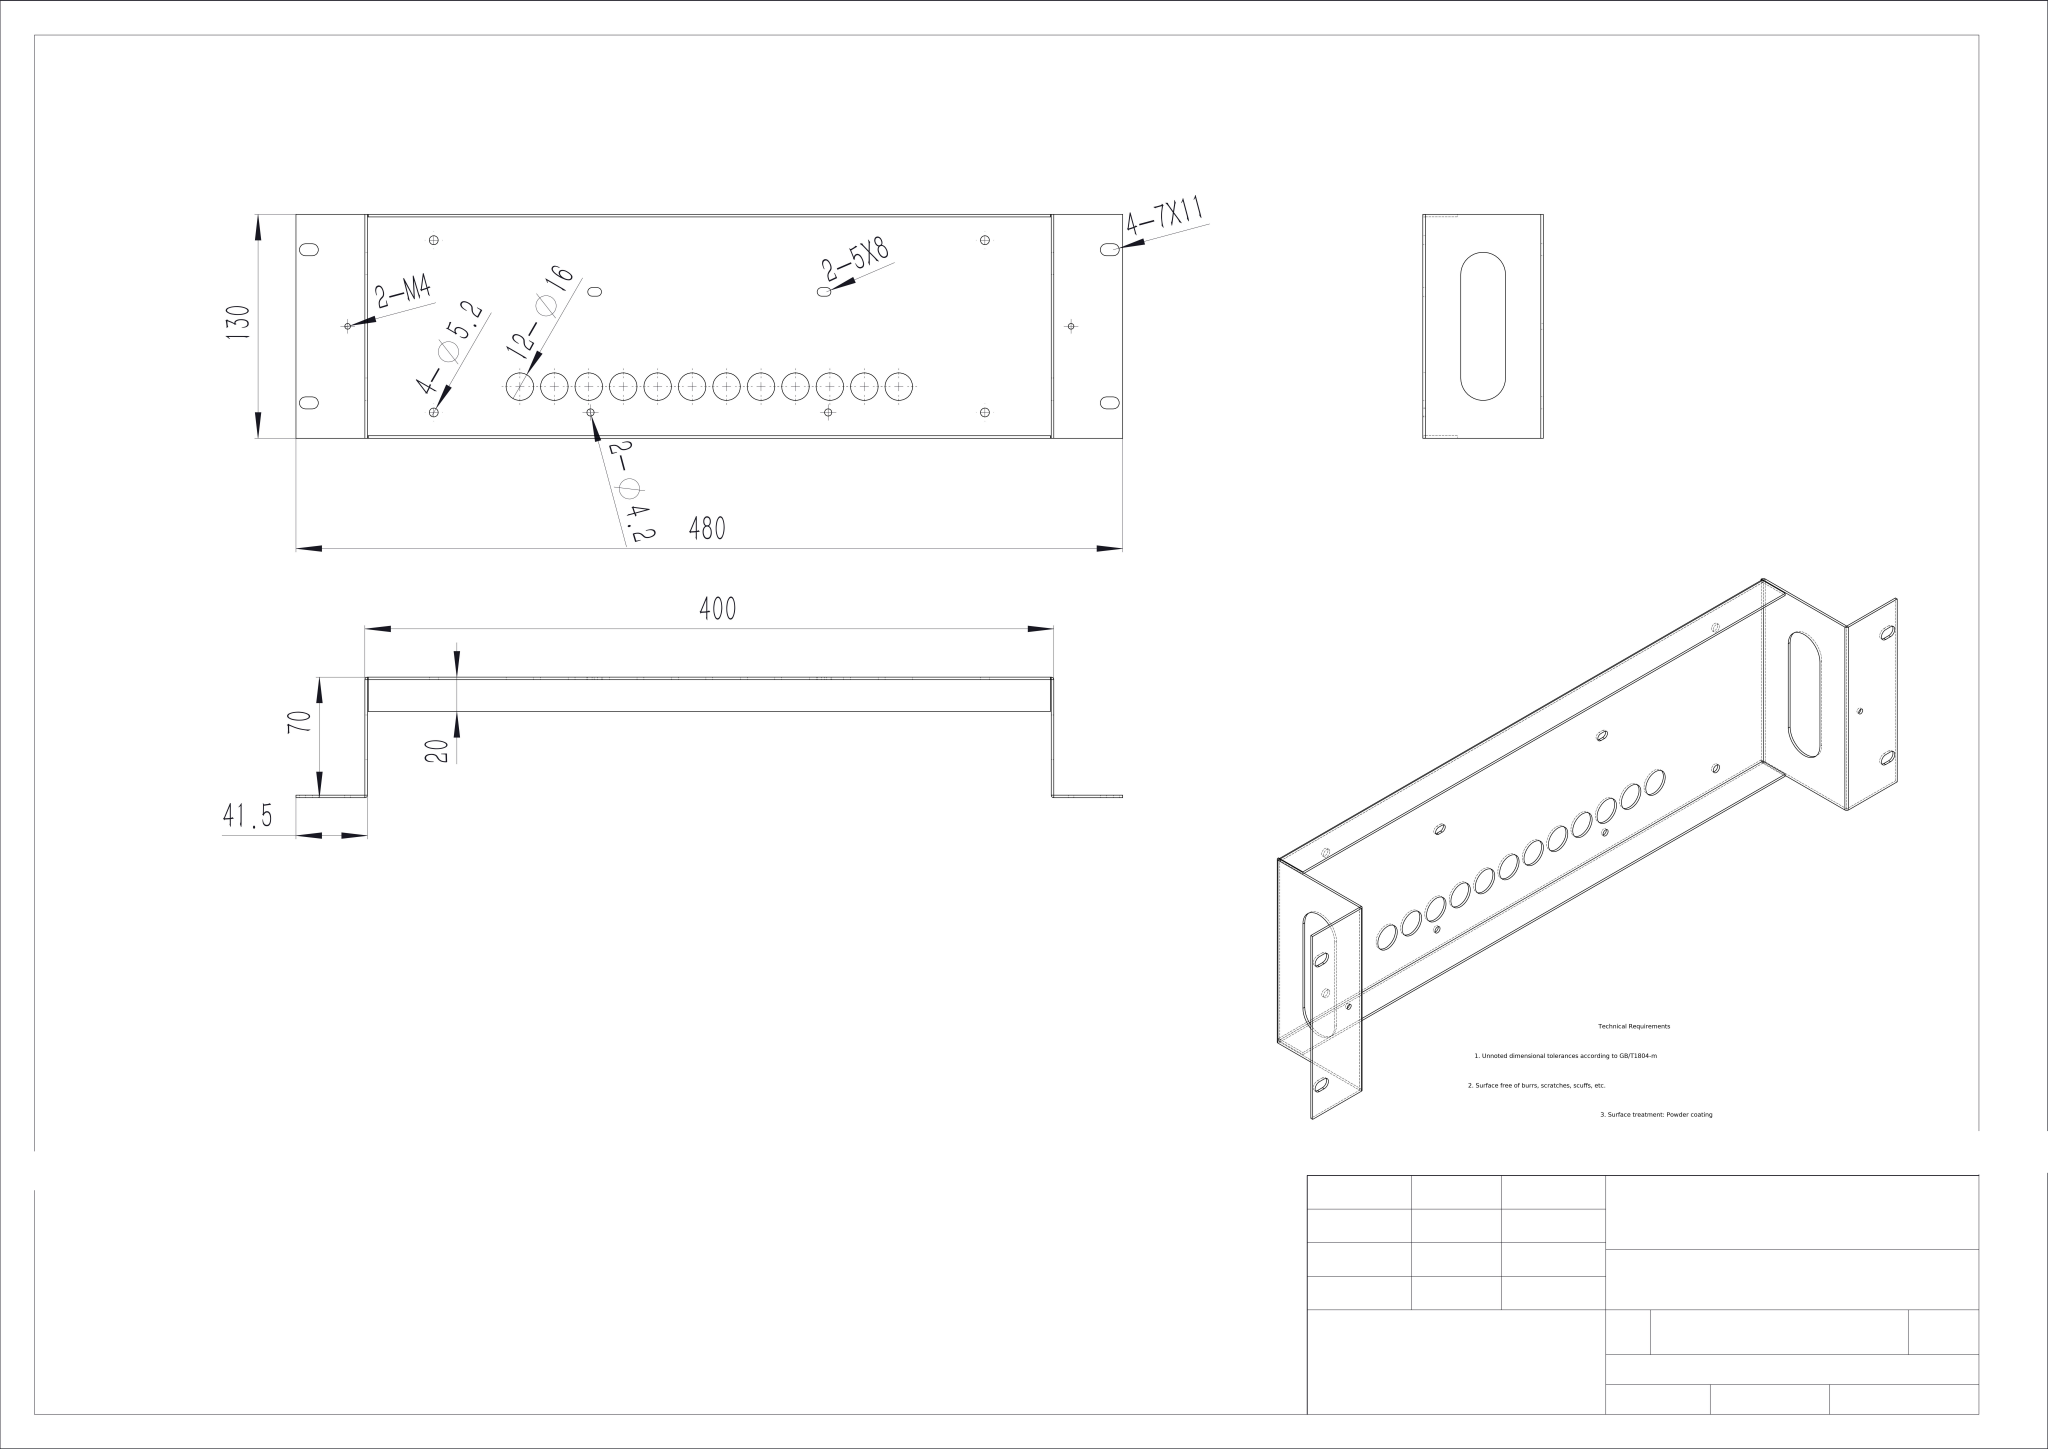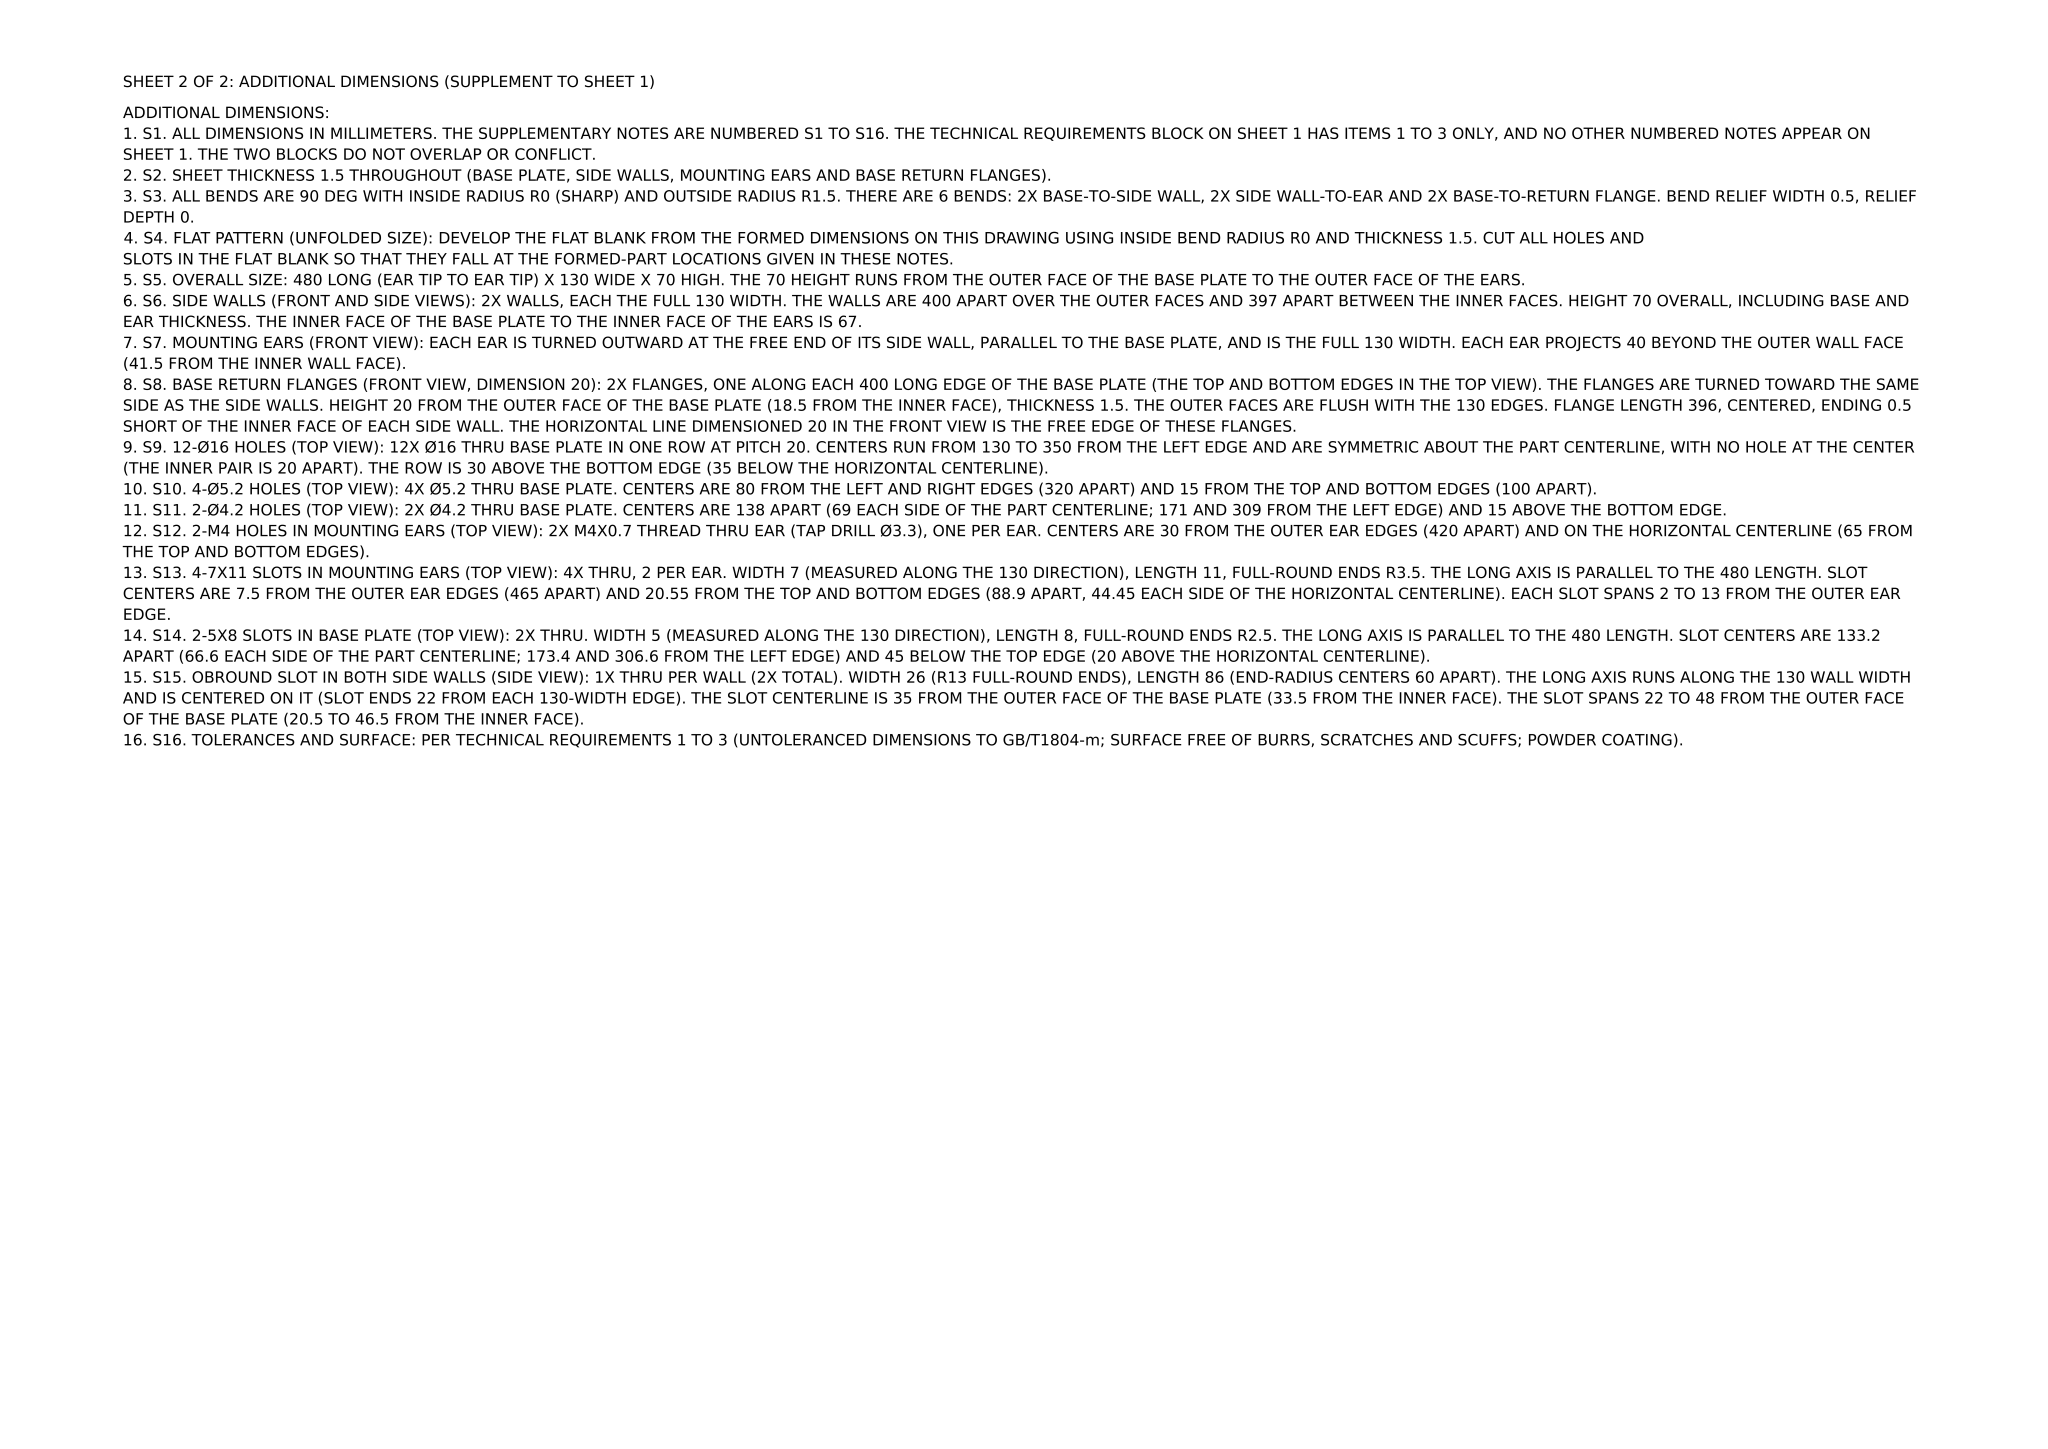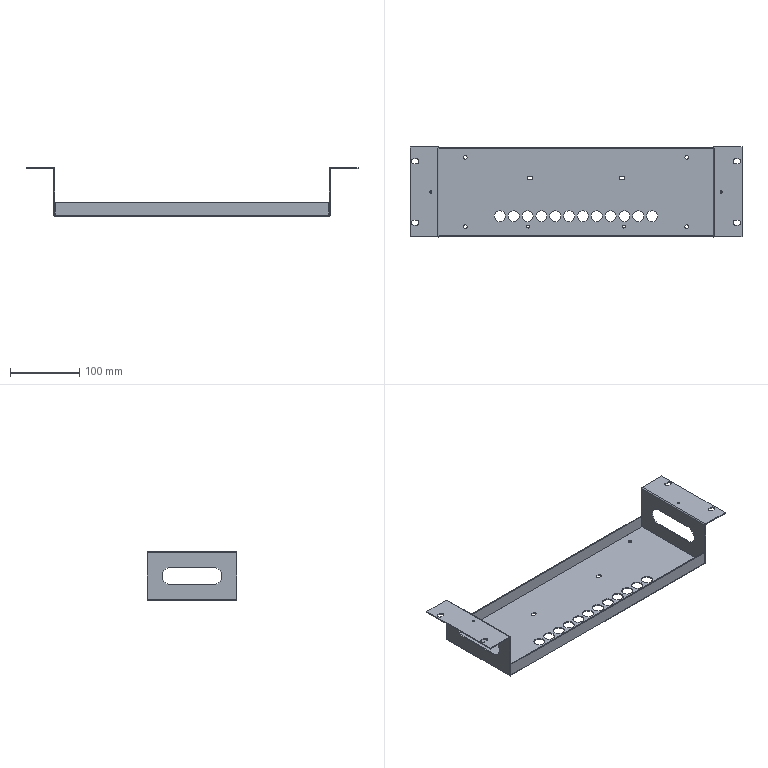Part | NX | mm | 1 solid | 148 faces | box 480 x 130 x 70 mm | volume 131069 mm3 | cylinder 74 | plane 74 | commonest cylinder face diameters 16 x24 7 x12 5.2 x8 5 x6 3.002 x6 0.002 x6 3.3 x4 4.2 x4